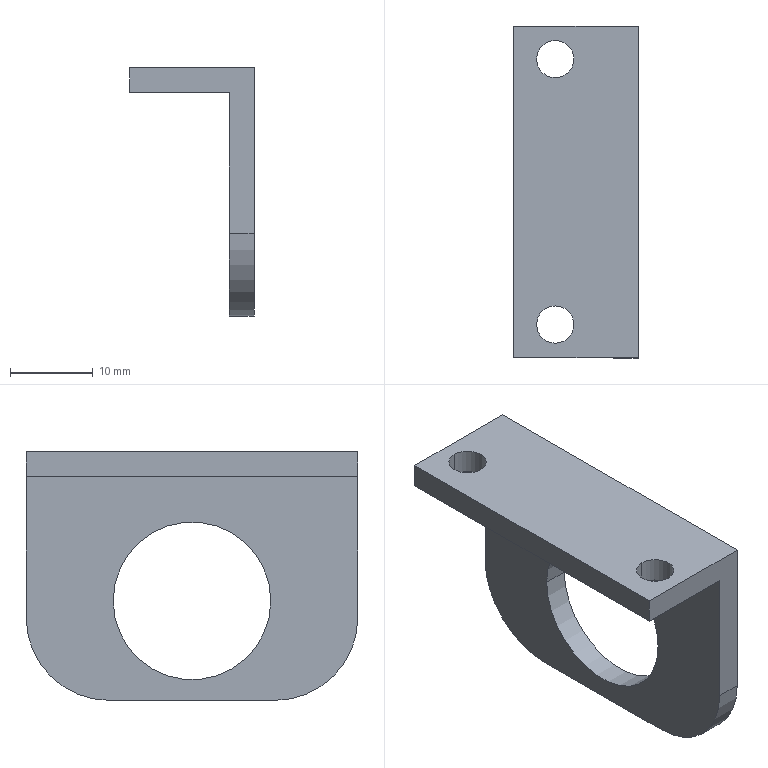Component | SolidWorks | 000-11-1 | 1 solid | 16 faces | box 15 x 40 x 30 mm | volume 3965 mm3 | cylinder 8 | plane 8 | commonest cylinder face diameters 4.5 x4 19 x2 20 x2 | material 6061
build123d program:
from build123d import *

# Parameters (mm, degrees)
SKETCH1_W           = 30
SKETCH1_H           = 15
BOSS_EXTRUDE1_DEPTH = 20
SKETCH2_W           = 27
SKETCH2_H           = 12
CUT_EXTRUDE1_DEPTH  = 44.373
SKETCH3_R           = 9.5
CUT_EXTRUDE2_DEPTH  = 30.155
FILLET1_R           = 10


with BuildPart() as part:
    # Sketch1 → Boss-Extrude1 (new, symmetric)
    with BuildSketch(Plane.XY):
        Rectangle(SKETCH1_W, SKETCH1_H)
    extrude(amount=BOSS_EXTRUDE1_DEPTH, both=True)

    # Sketch2 → Cut-Extrude1 (cut, through all)
    with BuildSketch(Plane.XY.offset(20)):
        with Locations((1.5, 1.5)):
            Rectangle(SKETCH2_W, SKETCH2_H)
    extrude(amount=-CUT_EXTRUDE1_DEPTH, mode=Mode.SUBTRACT)

    # Sketch3 → Cut-Extrude2 (cut, through all)
    with BuildSketch(Plane.XZ.offset(7.5)):
        with Locations(Location((3, 0, 0), (0, 0, 270))):
            Circle(SKETCH3_R)
    extrude(amount=-CUT_EXTRUDE2_DEPTH, mode=Mode.SUBTRACT)

    # Sketch5 → M4 Clearance Hole1 (revolve, cut)
    with BuildSketch(Plane(origin=(-12, 2.5, 16), x_dir=(0, 0, -1), z_dir=(0, 1, 0))):
        Polygon((0, 0), (0, 13.752), (2.25, 12.4), (2.25, 0), align=None)
    m4_clearance_hole1 = revolve(axis=Axis((-5.65, 2.5, 16), (-1, 0, 0)), mode=Mode.SUBTRACT)

    # Mirror1: M4 Clearance Hole1 across plane
    add(m4_clearance_hole1.mirror(Plane.XY), mode=Mode.SUBTRACT)

    # Fillet1
    fillet1_edges = [part.edges().sort_by_distance(p)[0] for p in [
        (15, -6, 20),
        (15, -6, -20),
    ]]
    fillet(fillet1_edges, radius=FILLET1_R)


solid = part.part

# Placed as in the assembly
solid = solid.moved(Location((171.5, 767, -140), (-90, 0, 90)))
STEP:
#1=COLOUR_RGB('',0.7922,0.8196,0.9333);
#2=FILL_AREA_STYLE_COLOUR('',#1);
#3=FILL_AREA_STYLE('',(#2));
#4=SURFACE_STYLE_FILL_AREA(#3);
#5=SURFACE_SIDE_STYLE('',(#4));
#6=SURFACE_STYLE_USAGE(.BOTH.,#5);
#7=PRESENTATION_STYLE_ASSIGNMENT((#6));
#8=CARTESIAN_POINT('',(6.654,29.656,-4.921));
#9=VERTEX_POINT('',#8);
#10=CARTESIAN_POINT('',(6.654,29.478,-4.921));
#11=VERTEX_POINT('',#10);
#12=CARTESIAN_POINT('',(6.654,29.567,-4.921));
#13=DIRECTION('',(-0.,0.,-1.));
#14=DIRECTION('',(0.,-1.,0.));
#15=AXIS2_PLACEMENT_3D('',#12,#13,#14);
#16=CIRCLE('',#15,0.08858);
#17=EDGE_CURVE('',#9,#11,#16,.T.);
#18=ORIENTED_EDGE('',*,*,#17,.F.);
#19=CARTESIAN_POINT('',(6.654,29.656,-5.039));
#20=VERTEX_POINT('',#19);
#21=CARTESIAN_POINT('',(6.654,29.656,-5.039));
#22=DIRECTION('',(-0.,0.,-1.));
#23=VECTOR('',#22,39.37);
#24=LINE('',#21,#23);
#25=EDGE_CURVE('',#9,#20,#24,.T.);
#26=ORIENTED_EDGE('',*,*,#25,.T.);
#27=CARTESIAN_POINT('',(6.654,29.478,-5.039));
#28=VERTEX_POINT('',#27);
#29=CARTESIAN_POINT('',(6.654,29.567,-5.039));
#30=DIRECTION('',(-0.,0.,-1.));
#31=DIRECTION('',(0.,-1.,0.));
#32=AXIS2_PLACEMENT_3D('',#29,#30,#31);
#33=CIRCLE('',#32,0.08858);
#34=EDGE_CURVE('',#20,#28,#33,.T.);
#35=ORIENTED_EDGE('',*,*,#34,.T.);
#36=CARTESIAN_POINT('',(6.654,29.478,-5.039));
#37=DIRECTION('',(-0.,0.,-1.));
#38=VECTOR('',#37,39.37);
#39=LINE('',#36,#38);
#40=EDGE_CURVE('',#11,#28,#39,.T.);
#41=ORIENTED_EDGE('',*,*,#40,.F.);
#42=EDGE_LOOP('',(#18,#26,#35,#41));
#43=FACE_OUTER_BOUND('',#42,.T.);
#44=CARTESIAN_POINT('',(6.654,29.567,-5.039));
#45=DIRECTION('',(-0.,0.,-1.));
#46=DIRECTION('',(0.,-1.,0.));
#47=AXIS2_PLACEMENT_3D('',#44,#45,#46);
#48=CYLINDRICAL_SURFACE('',#47,0.08858);
#49=ADVANCED_FACE('',(#43),#48,.F.);
#50=CARTESIAN_POINT('',(6.654,30.915,-4.921));
#51=VERTEX_POINT('',#50);
#52=CARTESIAN_POINT('',(6.654,30.738,-4.921));
#53=VERTEX_POINT('',#52);
#54=CARTESIAN_POINT('',(6.654,30.827,-4.921));
#55=DIRECTION('',(-0.,0.,-1.));
#56=DIRECTION('',(0.,-1.,0.));
#57=AXIS2_PLACEMENT_3D('',#54,#55,#56);
#58=CIRCLE('',#57,0.08858);
#59=EDGE_CURVE('',#51,#53,#58,.T.);
#60=ORIENTED_EDGE('',*,*,#59,.F.);
#61=CARTESIAN_POINT('',(6.654,30.915,-5.039));
#62=VERTEX_POINT('',#61);
#63=CARTESIAN_POINT('',(6.654,30.915,-5.039));
#64=DIRECTION('',(-0.,0.,-1.));
#65=VECTOR('',#64,39.37);
#66=LINE('',#63,#65);
#67=EDGE_CURVE('',#51,#62,#66,.T.);
#68=ORIENTED_EDGE('',*,*,#67,.T.);
#69=CARTESIAN_POINT('',(6.654,30.738,-5.039));
#70=VERTEX_POINT('',#69);
#71=CARTESIAN_POINT('',(6.654,30.827,-5.039));
#72=DIRECTION('',(-0.,0.,-1.));
#73=DIRECTION('',(0.,-1.,0.));
#74=AXIS2_PLACEMENT_3D('',#71,#72,#73);
#75=CIRCLE('',#74,0.08858);
#76=EDGE_CURVE('',#62,#70,#75,.T.);
#77=ORIENTED_EDGE('',*,*,#76,.T.);
#78=CARTESIAN_POINT('',(6.654,30.738,-5.039));
#79=DIRECTION('',(-0.,0.,-1.));
#80=VECTOR('',#79,39.37);
#81=LINE('',#78,#80);
#82=EDGE_CURVE('',#53,#70,#81,.T.);
#83=ORIENTED_EDGE('',*,*,#82,.F.);
#84=EDGE_LOOP('',(#60,#68,#77,#83));
#85=FACE_OUTER_BOUND('',#84,.T.);
#86=CARTESIAN_POINT('',(6.654,30.827,-5.039));
#87=DIRECTION('',(-0.,0.,-1.));
#88=DIRECTION('',(0.,-1.,0.));
#89=AXIS2_PLACEMENT_3D('',#86,#87,#88);
#90=CYLINDRICAL_SURFACE('',#89,0.08858);
#91=ADVANCED_FACE('',(#85),#90,.F.);
#92=CARTESIAN_POINT('',(6.929,30.571,-5.63));
#93=VERTEX_POINT('',#92);
#94=CARTESIAN_POINT('',(6.929,29.823,-5.63));
#95=VERTEX_POINT('',#94);
#96=CARTESIAN_POINT('',(6.929,30.197,-5.63));
#97=DIRECTION('',(1.,-0.,-0.));
#98=DIRECTION('',(0.,0.,-1.));
#99=AXIS2_PLACEMENT_3D('',#96,#97,#98);
#100=CIRCLE('',#99,0.374);
#101=EDGE_CURVE('',#93,#95,#100,.T.);
#102=ORIENTED_EDGE('',*,*,#101,.F.);
#103=CARTESIAN_POINT('',(7.047,30.571,-5.63));
#104=VERTEX_POINT('',#103);
#105=CARTESIAN_POINT('',(6.457,30.571,-5.63));
#106=DIRECTION('',(1.,-0.,-0.));
#107=VECTOR('',#106,39.37);
#108=LINE('',#105,#107);
#109=EDGE_CURVE('',#93,#104,#108,.T.);
#110=ORIENTED_EDGE('',*,*,#109,.T.);
#111=CARTESIAN_POINT('',(7.047,29.823,-5.63));
#112=VERTEX_POINT('',#111);
#113=CARTESIAN_POINT('',(7.047,30.197,-5.63));
#114=DIRECTION('',(1.,-0.,-0.));
#115=DIRECTION('',(0.,-1.,0.));
#116=AXIS2_PLACEMENT_3D('',#113,#114,#115);
#117=CIRCLE('',#116,0.374);
#118=EDGE_CURVE('',#104,#112,#117,.T.);
#119=ORIENTED_EDGE('',*,*,#118,.T.);
#120=CARTESIAN_POINT('',(6.457,29.823,-5.63));
#121=DIRECTION('',(1.,-0.,-0.));
#122=VECTOR('',#121,39.37);
#123=LINE('',#120,#122);
#124=EDGE_CURVE('',#95,#112,#123,.T.);
#125=ORIENTED_EDGE('',*,*,#124,.F.);
#126=EDGE_LOOP('',(#102,#110,#119,#125));
#127=FACE_OUTER_BOUND('',#126,.T.);
#128=CARTESIAN_POINT('',(6.457,30.197,-5.63));
#129=DIRECTION('',(1.,-0.,-0.));
#130=DIRECTION('',(0.,-1.,0.));
#131=AXIS2_PLACEMENT_3D('',#128,#129,#130);
#132=CYLINDRICAL_SURFACE('',#131,0.374);
#133=ADVANCED_FACE('',(#127),#132,.F.);
#134=CARTESIAN_POINT('',(7.047,30.591,-6.102));
#135=VERTEX_POINT('',#134);
#136=CARTESIAN_POINT('',(7.047,29.803,-6.102));
#137=VERTEX_POINT('',#136);
#138=CARTESIAN_POINT('',(7.047,30.984,-6.102));
#139=DIRECTION('',(-0.,-1.,-0.));
#140=VECTOR('',#139,39.37);
#141=LINE('',#138,#140);
#142=EDGE_CURVE('',#135,#137,#141,.T.);
#143=ORIENTED_EDGE('',*,*,#142,.T.);
#144=CARTESIAN_POINT('',(6.929,29.803,-6.102));
#145=VERTEX_POINT('',#144);
#146=CARTESIAN_POINT('',(6.929,29.803,-6.102));
#147=DIRECTION('',(-1.,0.,0.));
#148=VECTOR('',#147,39.37);
#149=LINE('',#146,#148);
#150=EDGE_CURVE('',#137,#145,#149,.T.);
#151=ORIENTED_EDGE('',*,*,#150,.T.);
#152=CARTESIAN_POINT('',(6.929,30.591,-6.102));
#153=VERTEX_POINT('',#152);
#154=CARTESIAN_POINT('',(6.929,29.409,-6.102));
#155=DIRECTION('',(0.,1.,0.));
#156=VECTOR('',#155,39.37);
#157=LINE('',#154,#156);
#158=EDGE_CURVE('',#145,#153,#157,.T.);
#159=ORIENTED_EDGE('',*,*,#158,.T.);
#160=CARTESIAN_POINT('',(7.047,30.591,-6.102));
#161=DIRECTION('',(1.,-0.,-0.));
#162=VECTOR('',#161,39.37);
#163=LINE('',#160,#162);
#164=EDGE_CURVE('',#153,#135,#163,.T.);
#165=ORIENTED_EDGE('',*,*,#164,.T.);
#166=EDGE_LOOP('',(#143,#151,#159,#165));
#167=FACE_OUTER_BOUND('',#166,.T.);
#168=CARTESIAN_POINT('',(7.047,30.984,-6.102));
#169=DIRECTION('',(0.,-0.,1.));
#170=DIRECTION('',(0.,1.,0.));
#171=AXIS2_PLACEMENT_3D('',#168,#169,#170);
#172=PLANE('',#171);
#173=ADVANCED_FACE('',(#167),#172,.F.);
#174=CARTESIAN_POINT('',(6.457,30.984,-5.039));
#175=VERTEX_POINT('',#174);
#176=CARTESIAN_POINT('',(6.457,30.984,-4.921));
#177=VERTEX_POINT('',#176);
#178=CARTESIAN_POINT('',(6.457,30.984,-4.921));
#179=DIRECTION('',(0.,-0.,1.));
#180=VECTOR('',#179,39.37);
#181=LINE('',#178,#180);
#182=EDGE_CURVE('',#175,#177,#181,.T.);
#183=ORIENTED_EDGE('',*,*,#182,.F.);
#184=CARTESIAN_POINT('',(6.457,29.409,-5.039));
#185=VERTEX_POINT('',#184);
#186=CARTESIAN_POINT('',(6.457,29.409,-5.039));
#187=DIRECTION('',(0.,1.,0.));
#188=VECTOR('',#187,39.37);
#189=LINE('',#186,#188);
#190=EDGE_CURVE('',#185,#175,#189,.T.);
#191=ORIENTED_EDGE('',*,*,#190,.F.);
#192=CARTESIAN_POINT('',(6.457,29.409,-4.921));
#193=VERTEX_POINT('',#192);
#194=CARTESIAN_POINT('',(6.457,29.409,-4.921));
#195=DIRECTION('',(0.,-0.,1.));
#196=VECTOR('',#195,39.37);
#197=LINE('',#194,#196);
#198=EDGE_CURVE('',#185,#193,#197,.T.);
#199=ORIENTED_EDGE('',*,*,#198,.T.);
#200=CARTESIAN_POINT('',(6.457,30.984,-4.921));
#201=DIRECTION('',(-0.,-1.,-0.));
#202=VECTOR('',#201,39.37);
#203=LINE('',#200,#202);
#204=EDGE_CURVE('',#177,#193,#203,.T.);
#205=ORIENTED_EDGE('',*,*,#204,.F.);
#206=EDGE_LOOP('',(#183,#191,#199,#205));
#207=FACE_OUTER_BOUND('',#206,.T.);
#208=CARTESIAN_POINT('',(6.457,30.984,-4.921));
#209=DIRECTION('',(1.,-0.,-0.));
#210=DIRECTION('',(-0.,-1.,-0.));
#211=AXIS2_PLACEMENT_3D('',#208,#209,#210);
#212=PLANE('',#211);
#213=ADVANCED_FACE('',(#207),#212,.F.);
#214=CARTESIAN_POINT('',(6.654,29.567,-4.921));
#215=DIRECTION('',(-0.,0.,-1.));
#216=DIRECTION('',(0.,-1.,0.));
#217=AXIS2_PLACEMENT_3D('',#214,#215,#216);
#218=CIRCLE('',#217,0.08858);
#219=EDGE_CURVE('',#11,#9,#218,.T.);
#220=ORIENTED_EDGE('',*,*,#219,.T.);
#221=ORIENTED_EDGE('',*,*,#17,.T.);
#222=EDGE_LOOP('',(#220,#221));
#223=FACE_BOUND('',#222,.T.);
#224=CARTESIAN_POINT('',(6.654,30.827,-4.921));
#225=DIRECTION('',(-0.,0.,-1.));
#226=DIRECTION('',(0.,-1.,0.));
#227=AXIS2_PLACEMENT_3D('',#224,#225,#226);
#228=CIRCLE('',#227,0.08858);
#229=EDGE_CURVE('',#53,#51,#228,.T.);
#230=ORIENTED_EDGE('',*,*,#229,.T.);
#231=ORIENTED_EDGE('',*,*,#59,.T.);
#232=EDGE_LOOP('',(#230,#231));
#233=FACE_BOUND('',#232,.T.);
#234=CARTESIAN_POINT('',(7.047,29.409,-4.921));
#235=VERTEX_POINT('',#234);
#236=CARTESIAN_POINT('',(7.047,29.409,-4.921));
#237=DIRECTION('',(1.,-0.,-0.));
#238=VECTOR('',#237,39.37);
#239=LINE('',#236,#238);
#240=EDGE_CURVE('',#193,#235,#239,.T.);
#241=ORIENTED_EDGE('',*,*,#240,.T.);
#242=CARTESIAN_POINT('',(7.047,30.984,-4.921));
#243=VERTEX_POINT('',#242);
#244=CARTESIAN_POINT('',(7.047,30.984,-4.921));
#245=DIRECTION('',(-0.,-1.,-0.));
#246=VECTOR('',#245,39.37);
#247=LINE('',#244,#246);
#248=EDGE_CURVE('',#243,#235,#247,.T.);
#249=ORIENTED_EDGE('',*,*,#248,.F.);
#250=CARTESIAN_POINT('',(7.047,30.984,-4.921));
#251=DIRECTION('',(1.,-0.,-0.));
#252=VECTOR('',#251,39.37);
#253=LINE('',#250,#252);
#254=EDGE_CURVE('',#177,#243,#253,.T.);
#255=ORIENTED_EDGE('',*,*,#254,.F.);
#256=ORIENTED_EDGE('',*,*,#204,.T.);
#257=EDGE_LOOP('',(#241,#249,#255,#256));
#258=FACE_OUTER_BOUND('',#257,.T.);
#259=CARTESIAN_POINT('',(7.047,30.984,-4.921));
#260=DIRECTION('',(-0.,0.,-1.));
#261=DIRECTION('',(-0.,-1.,-0.));
#262=AXIS2_PLACEMENT_3D('',#259,#260,#261);
#263=PLANE('',#262);
#264=ADVANCED_FACE('',(#223,#233,#258),#263,.F.);
#265=CARTESIAN_POINT('',(7.047,30.197,-5.63));
#266=DIRECTION('',(1.,-0.,-0.));
#267=DIRECTION('',(0.,-1.,0.));
#268=AXIS2_PLACEMENT_3D('',#265,#266,#267);
#269=CIRCLE('',#268,0.374);
#270=EDGE_CURVE('',#112,#104,#269,.T.);
#271=ORIENTED_EDGE('',*,*,#270,.F.);
#272=ORIENTED_EDGE('',*,*,#118,.F.);
#273=EDGE_LOOP('',(#271,#272));
#274=FACE_BOUND('',#273,.T.);
#275=CARTESIAN_POINT('',(7.047,29.409,-5.709));
#276=VERTEX_POINT('',#275);
#277=CARTESIAN_POINT('',(7.047,29.409,-4.921));
#278=DIRECTION('',(-0.,0.,-1.));
#279=VECTOR('',#278,39.37);
#280=LINE('',#277,#279);
#281=EDGE_CURVE('',#235,#276,#280,.T.);
#282=ORIENTED_EDGE('',*,*,#281,.T.);
#283=CARTESIAN_POINT('',(7.047,29.803,-5.709));
#284=DIRECTION('',(1.,-0.,-0.));
#285=DIRECTION('',(0.,1.,0.));
#286=AXIS2_PLACEMENT_3D('',#283,#284,#285);
#287=CIRCLE('',#286,0.3937);
#288=EDGE_CURVE('',#276,#137,#287,.T.);
#289=ORIENTED_EDGE('',*,*,#288,.T.);
#290=ORIENTED_EDGE('',*,*,#142,.F.);
#291=CARTESIAN_POINT('',(7.047,30.984,-5.709));
#292=VERTEX_POINT('',#291);
#293=CARTESIAN_POINT('',(7.047,30.591,-5.709));
#294=DIRECTION('',(1.,-0.,-0.));
#295=DIRECTION('',(0.,1.,-0.));
#296=AXIS2_PLACEMENT_3D('',#293,#294,#295);
#297=CIRCLE('',#296,0.3937);
#298=EDGE_CURVE('',#135,#292,#297,.T.);
#299=ORIENTED_EDGE('',*,*,#298,.T.);
#300=CARTESIAN_POINT('',(7.047,30.984,-4.921));
#301=DIRECTION('',(-0.,0.,-1.));
#302=VECTOR('',#301,39.37);
#303=LINE('',#300,#302);
#304=EDGE_CURVE('',#243,#292,#303,.T.);
#305=ORIENTED_EDGE('',*,*,#304,.F.);
#306=ORIENTED_EDGE('',*,*,#248,.T.);
#307=EDGE_LOOP('',(#282,#289,#290,#299,#305,#306));
#308=FACE_OUTER_BOUND('',#307,.T.);
#309=CARTESIAN_POINT('',(7.047,30.984,-4.921));
#310=DIRECTION('',(-1.,0.,0.));
#311=DIRECTION('',(0.,1.,0.));
#312=AXIS2_PLACEMENT_3D('',#309,#310,#311);
#313=PLANE('',#312);
#314=ADVANCED_FACE('',(#274,#308),#313,.F.);
#315=ORIENTED_EDGE('',*,*,#304,.T.);
#316=CARTESIAN_POINT('',(6.929,30.984,-5.709));
#317=VERTEX_POINT('',#316);
#318=CARTESIAN_POINT('',(6.752,30.984,-5.709));
#319=DIRECTION('',(-1.,0.,0.));
#320=VECTOR('',#319,39.37);
#321=LINE('',#318,#320);
#322=EDGE_CURVE('',#292,#317,#321,.T.);
#323=ORIENTED_EDGE('',*,*,#322,.T.);
#324=CARTESIAN_POINT('',(6.929,30.984,-5.039));
#325=VERTEX_POINT('',#324);
#326=CARTESIAN_POINT('',(6.929,30.984,-6.102));
#327=DIRECTION('',(-0.,0.,-1.));
#328=VECTOR('',#327,39.37);
#329=LINE('',#326,#328);
#330=EDGE_CURVE('',#325,#317,#329,.T.);
#331=ORIENTED_EDGE('',*,*,#330,.F.);
#332=CARTESIAN_POINT('',(6.457,30.984,-5.039));
#333=DIRECTION('',(1.,-0.,-0.));
#334=VECTOR('',#333,39.37);
#335=LINE('',#332,#334);
#336=EDGE_CURVE('',#175,#325,#335,.T.);
#337=ORIENTED_EDGE('',*,*,#336,.F.);
#338=ORIENTED_EDGE('',*,*,#182,.T.);
#339=ORIENTED_EDGE('',*,*,#254,.T.);
#340=EDGE_LOOP('',(#315,#323,#331,#337,#338,#339));
#341=FACE_OUTER_BOUND('',#340,.T.);
#342=CARTESIAN_POINT('',(6.752,30.984,-5.512));
#343=DIRECTION('',(-0.,-1.,-0.));
#344=DIRECTION('',(0.,-0.,1.));
#345=AXIS2_PLACEMENT_3D('',#342,#343,#344);
#346=PLANE('',#345);
#347=ADVANCED_FACE('',(#341),#346,.F.);
#348=CARTESIAN_POINT('',(6.929,29.409,-5.039));
#349=VERTEX_POINT('',#348);
#350=CARTESIAN_POINT('',(6.929,29.409,-5.709));
#351=VERTEX_POINT('',#350);
#352=CARTESIAN_POINT('',(6.929,29.409,-6.102));
#353=DIRECTION('',(-0.,0.,-1.));
#354=VECTOR('',#353,39.37);
#355=LINE('',#352,#354);
#356=EDGE_CURVE('',#349,#351,#355,.T.);
#357=ORIENTED_EDGE('',*,*,#356,.T.);
#358=CARTESIAN_POINT('',(7.047,29.409,-5.709));
#359=DIRECTION('',(1.,-0.,-0.));
#360=VECTOR('',#359,39.37);
#361=LINE('',#358,#360);
#362=EDGE_CURVE('',#351,#276,#361,.T.);
#363=ORIENTED_EDGE('',*,*,#362,.T.);
#364=ORIENTED_EDGE('',*,*,#281,.F.);
#365=ORIENTED_EDGE('',*,*,#240,.F.);
#366=ORIENTED_EDGE('',*,*,#198,.F.);
#367=CARTESIAN_POINT('',(6.457,29.409,-5.039));
#368=DIRECTION('',(1.,-0.,-0.));
#369=VECTOR('',#368,39.37);
#370=LINE('',#367,#369);
#371=EDGE_CURVE('',#185,#349,#370,.T.);
#372=ORIENTED_EDGE('',*,*,#371,.T.);
#373=EDGE_LOOP('',(#357,#363,#364,#365,#366,#372));
#374=FACE_OUTER_BOUND('',#373,.T.);
#375=CARTESIAN_POINT('',(6.752,29.409,-5.512));
#376=DIRECTION('',(-0.,-1.,-0.));
#377=DIRECTION('',(0.,-0.,1.));
#378=AXIS2_PLACEMENT_3D('',#375,#376,#377);
#379=PLANE('',#378);
#380=ADVANCED_FACE('',(#374),#379,.T.);
#381=CARTESIAN_POINT('',(6.929,30.197,-5.63));
#382=DIRECTION('',(1.,-0.,-0.));
#383=DIRECTION('',(0.,0.,-1.));
#384=AXIS2_PLACEMENT_3D('',#381,#382,#383);
#385=CIRCLE('',#384,0.374);
#386=EDGE_CURVE('',#95,#93,#385,.T.);
#387=ORIENTED_EDGE('',*,*,#386,.T.);
#388=ORIENTED_EDGE('',*,*,#101,.T.);
#389=EDGE_LOOP('',(#387,#388));
#390=FACE_BOUND('',#389,.T.);
#391=ORIENTED_EDGE('',*,*,#158,.F.);
#392=CARTESIAN_POINT('',(6.929,29.803,-5.709));
#393=DIRECTION('',(-1.,0.,0.));
#394=DIRECTION('',(0.,0.,-1.));
#395=AXIS2_PLACEMENT_3D('',#392,#393,#394);
#396=CIRCLE('',#395,0.3937);
#397=EDGE_CURVE('',#145,#351,#396,.T.);
#398=ORIENTED_EDGE('',*,*,#397,.T.);
#399=ORIENTED_EDGE('',*,*,#356,.F.);
#400=CARTESIAN_POINT('',(6.929,29.409,-5.039));
#401=DIRECTION('',(0.,1.,0.));
#402=VECTOR('',#401,39.37);
#403=LINE('',#400,#402);
#404=EDGE_CURVE('',#349,#325,#403,.T.);
#405=ORIENTED_EDGE('',*,*,#404,.T.);
#406=ORIENTED_EDGE('',*,*,#330,.T.);
#407=CARTESIAN_POINT('',(6.929,30.591,-5.709));
#408=DIRECTION('',(-1.,0.,0.));
#409=DIRECTION('',(0.,0.,-1.));
#410=AXIS2_PLACEMENT_3D('',#407,#408,#409);
#411=CIRCLE('',#410,0.3937);
#412=EDGE_CURVE('',#317,#153,#411,.T.);
#413=ORIENTED_EDGE('',*,*,#412,.T.);
#414=EDGE_LOOP('',(#391,#398,#399,#405,#406,#413));
#415=FACE_OUTER_BOUND('',#414,.T.);
#416=CARTESIAN_POINT('',(6.929,29.409,-6.102));
#417=DIRECTION('',(1.,-0.,-0.));
#418=DIRECTION('',(-0.,0.,-1.));
#419=AXIS2_PLACEMENT_3D('',#416,#417,#418);
#420=PLANE('',#419);
#421=ADVANCED_FACE('',(#390,#415),#420,.F.);
#422=CARTESIAN_POINT('',(6.654,29.567,-5.039));
#423=DIRECTION('',(-0.,0.,-1.));
#424=DIRECTION('',(0.,-1.,0.));
#425=AXIS2_PLACEMENT_3D('',#422,#423,#424);
#426=CIRCLE('',#425,0.08858);
#427=EDGE_CURVE('',#28,#20,#426,.T.);
#428=ORIENTED_EDGE('',*,*,#427,.F.);
#429=ORIENTED_EDGE('',*,*,#34,.F.);
#430=EDGE_LOOP('',(#428,#429));
#431=FACE_BOUND('',#430,.T.);
#432=CARTESIAN_POINT('',(6.654,30.827,-5.039));
#433=DIRECTION('',(-0.,0.,-1.));
#434=DIRECTION('',(0.,-1.,0.));
#435=AXIS2_PLACEMENT_3D('',#432,#433,#434);
#436=CIRCLE('',#435,0.08858);
#437=EDGE_CURVE('',#70,#62,#436,.T.);
#438=ORIENTED_EDGE('',*,*,#437,.F.);
#439=ORIENTED_EDGE('',*,*,#76,.F.);
#440=EDGE_LOOP('',(#438,#439));
#441=FACE_BOUND('',#440,.T.);
#442=ORIENTED_EDGE('',*,*,#336,.T.);
#443=ORIENTED_EDGE('',*,*,#404,.F.);
#444=ORIENTED_EDGE('',*,*,#371,.F.);
#445=ORIENTED_EDGE('',*,*,#190,.T.);
#446=EDGE_LOOP('',(#442,#443,#444,#445));
#447=FACE_OUTER_BOUND('',#446,.T.);
#448=CARTESIAN_POINT('',(6.457,29.409,-5.039));
#449=DIRECTION('',(0.,-0.,1.));
#450=DIRECTION('',(1.,-0.,-0.));
#451=AXIS2_PLACEMENT_3D('',#448,#449,#450);
#452=PLANE('',#451);
#453=ADVANCED_FACE('',(#431,#441,#447),#452,.F.);
#454=ORIENTED_EDGE('',*,*,#109,.F.);
#455=ORIENTED_EDGE('',*,*,#386,.F.);
#456=ORIENTED_EDGE('',*,*,#124,.T.);
#457=ORIENTED_EDGE('',*,*,#270,.T.);
#458=EDGE_LOOP('',(#454,#455,#456,#457));
#459=FACE_OUTER_BOUND('',#458,.T.);
#460=CARTESIAN_POINT('',(6.457,30.197,-5.63));
#461=DIRECTION('',(1.,-0.,-0.));
#462=DIRECTION('',(0.,-1.,0.));
#463=AXIS2_PLACEMENT_3D('',#460,#461,#462);
#464=CYLINDRICAL_SURFACE('',#463,0.374);
#465=ADVANCED_FACE('',(#459),#464,.F.);
#466=ORIENTED_EDGE('',*,*,#67,.F.);
#467=ORIENTED_EDGE('',*,*,#229,.F.);
#468=ORIENTED_EDGE('',*,*,#82,.T.);
#469=ORIENTED_EDGE('',*,*,#437,.T.);
#470=EDGE_LOOP('',(#466,#467,#468,#469));
#471=FACE_OUTER_BOUND('',#470,.T.);
#472=CARTESIAN_POINT('',(6.654,30.827,-5.039));
#473=DIRECTION('',(-0.,0.,-1.));
#474=DIRECTION('',(0.,-1.,0.));
#475=AXIS2_PLACEMENT_3D('',#472,#473,#474);
#476=CYLINDRICAL_SURFACE('',#475,0.08858);
#477=ADVANCED_FACE('',(#471),#476,.F.);
#478=ORIENTED_EDGE('',*,*,#25,.F.);
#479=ORIENTED_EDGE('',*,*,#219,.F.);
#480=ORIENTED_EDGE('',*,*,#40,.T.);
#481=ORIENTED_EDGE('',*,*,#427,.T.);
#482=EDGE_LOOP('',(#478,#479,#480,#481));
#483=FACE_OUTER_BOUND('',#482,.T.);
#484=CARTESIAN_POINT('',(6.654,29.567,-5.039));
#485=DIRECTION('',(-0.,0.,-1.));
#486=DIRECTION('',(0.,-1.,0.));
#487=AXIS2_PLACEMENT_3D('',#484,#485,#486);
#488=CYLINDRICAL_SURFACE('',#487,0.08858);
#489=ADVANCED_FACE('',(#483),#488,.F.);
#490=ORIENTED_EDGE('',*,*,#288,.F.);
#491=ORIENTED_EDGE('',*,*,#362,.F.);
#492=ORIENTED_EDGE('',*,*,#397,.F.);
#493=ORIENTED_EDGE('',*,*,#150,.F.);
#494=EDGE_LOOP('',(#490,#491,#492,#493));
#495=FACE_OUTER_BOUND('',#494,.T.);
#496=CARTESIAN_POINT('',(7.047,29.803,-5.709));
#497=DIRECTION('',(1.,-0.,-0.));
#498=DIRECTION('',(0.,-1.,0.));
#499=AXIS2_PLACEMENT_3D('',#496,#497,#498);
#500=CYLINDRICAL_SURFACE('',#499,0.3937);
#501=ADVANCED_FACE('',(#495),#500,.T.);
#502=ORIENTED_EDGE('',*,*,#298,.F.);
#503=ORIENTED_EDGE('',*,*,#164,.F.);
#504=ORIENTED_EDGE('',*,*,#412,.F.);
#505=ORIENTED_EDGE('',*,*,#322,.F.);
#506=EDGE_LOOP('',(#502,#503,#504,#505));
#507=FACE_OUTER_BOUND('',#506,.T.);
#508=CARTESIAN_POINT('',(6.752,30.591,-5.709));
#509=DIRECTION('',(-1.,0.,0.));
#510=DIRECTION('',(0.,1.,0.));
#511=AXIS2_PLACEMENT_3D('',#508,#509,#510);
#512=CYLINDRICAL_SURFACE('',#511,0.3937);
#513=ADVANCED_FACE('',(#507),#512,.T.);
#514=CLOSED_SHELL('',(#49,#91,#133,#173,#213,#264,#314,#347,#380,#421,#453,#465,#477,#489,#501,#513));
#515=MANIFOLD_SOLID_BREP('',#514);
#516=STYLED_ITEM('',(#7),#515);
#517=PRESENTATION_LAYER_ASSIGNMENT('','',(#516));
#518=(LENGTH_UNIT()NAMED_UNIT(*)SI_UNIT($,.METRE.));
#519=LENGTH_MEASURE_WITH_UNIT(LENGTH_MEASURE(0.0254),#518);
#520=DIMENSIONAL_EXPONENTS(1.,0.,0.,0.,0.,0.,0.);
#521=(CONVERSION_BASED_UNIT('',#519)LENGTH_UNIT()NAMED_UNIT(#520));
#522=UNCERTAINTY_MEASURE_WITH_UNIT(LENGTH_MEASURE(0.00001),#521,'','');
#523=(NAMED_UNIT(*)PLANE_ANGLE_UNIT()SI_UNIT($,.RADIAN.));
#524=(NAMED_UNIT(*)SI_UNIT($,.STERADIAN.)SOLID_ANGLE_UNIT());
#525=(GEOMETRIC_REPRESENTATION_CONTEXT(3)GLOBAL_UNCERTAINTY_ASSIGNED_CONTEXT((#522))GLOBAL_UNIT_ASSIGNED_CONTEXT((#521,#523,#524))REPRESENTATION_CONTEXT('',''));
#526=MECHANICAL_DESIGN_GEOMETRIC_PRESENTATION_REPRESENTATION('',(#516),#525);
#527=CARTESIAN_POINT('',(0.,0.,0.));
#528=DIRECTION('',(0.,0.,1.));
#529=DIRECTION('',(1.,0.,0.));
#530=AXIS2_PLACEMENT_3D('',#527,#528,#529);
#531=(LENGTH_UNIT()NAMED_UNIT(*)SI_UNIT($,.METRE.));
#532=LENGTH_MEASURE_WITH_UNIT(LENGTH_MEASURE(0.0254),#531);
#533=DIMENSIONAL_EXPONENTS(1.,0.,0.,0.,0.,0.,0.);
#534=(CONVERSION_BASED_UNIT('',#532)LENGTH_UNIT()NAMED_UNIT(#533));
#535=UNCERTAINTY_MEASURE_WITH_UNIT(LENGTH_MEASURE(0.00001),#534,'','');
#536=(NAMED_UNIT(*)PLANE_ANGLE_UNIT()SI_UNIT($,.RADIAN.));
#537=(NAMED_UNIT(*)SI_UNIT($,.STERADIAN.)SOLID_ANGLE_UNIT());
#538=(GEOMETRIC_REPRESENTATION_CONTEXT(3)GLOBAL_UNCERTAINTY_ASSIGNED_CONTEXT((#535))GLOBAL_UNIT_ASSIGNED_CONTEXT((#534,#536,#537))REPRESENTATION_CONTEXT('',''));
#539=ADVANCED_BREP_SHAPE_REPRESENTATION('',(#515,#530),#538);